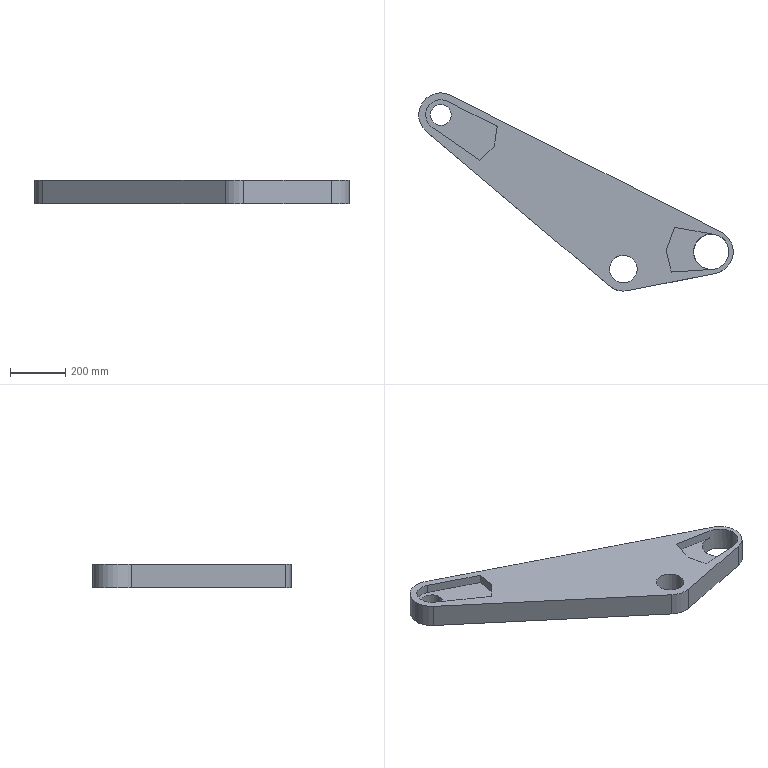Component | NX | TRI_ARM | 1 solid | 22 faces | volume 23133975 mm3 | plane 15 | cylinder 7 | commonest cylinder face diameters 160 x3 110 x1 128 x1 100 x1 76 x1